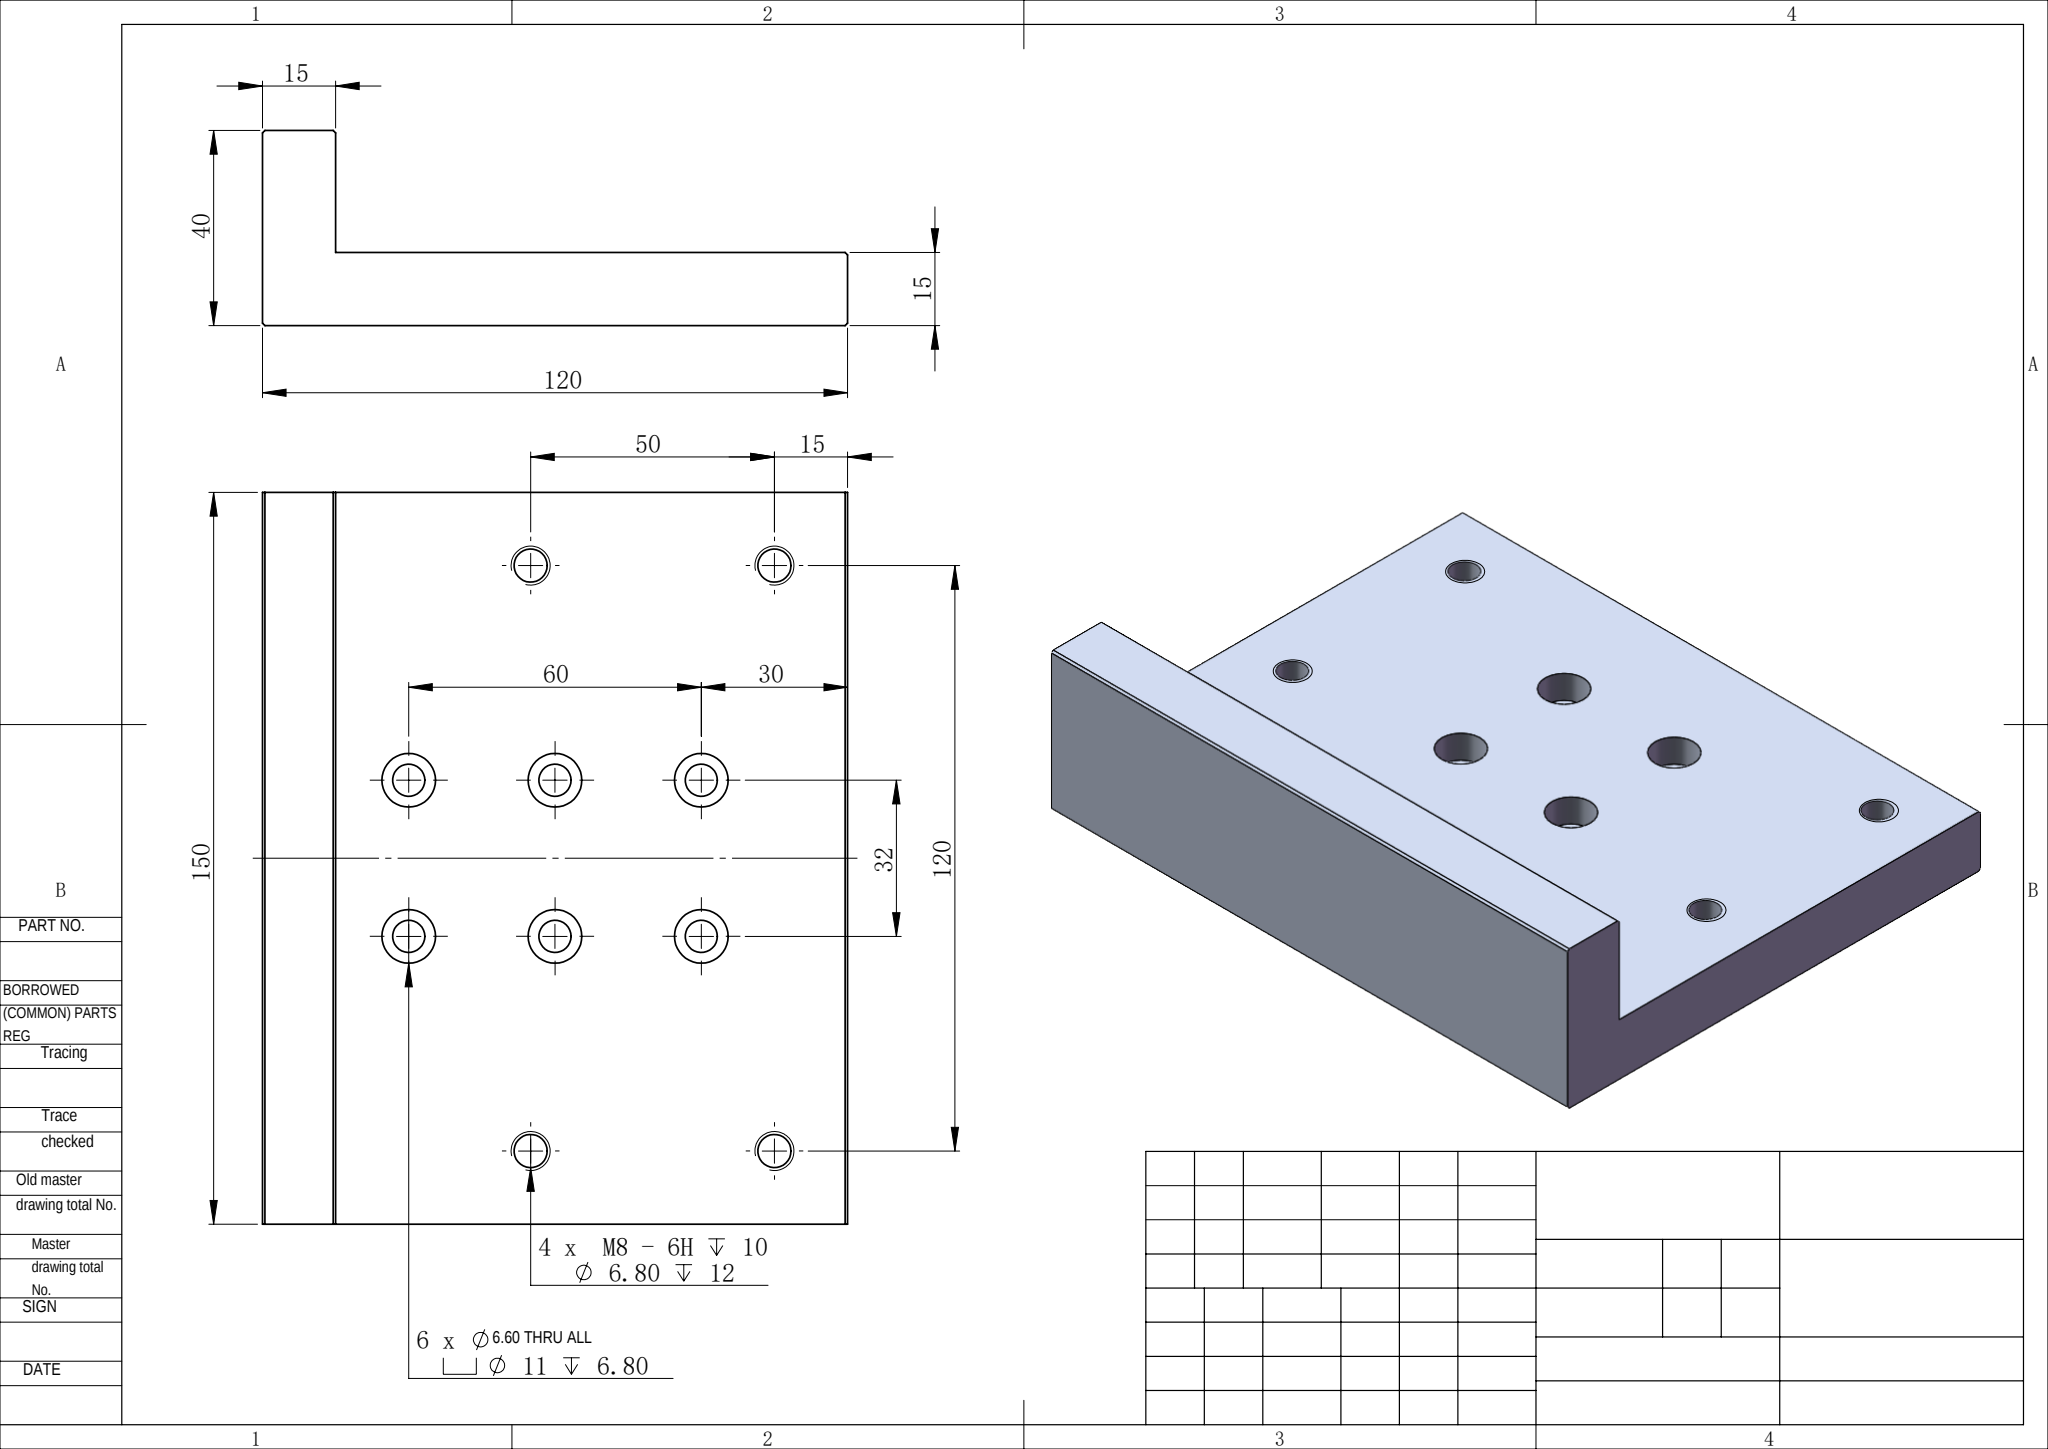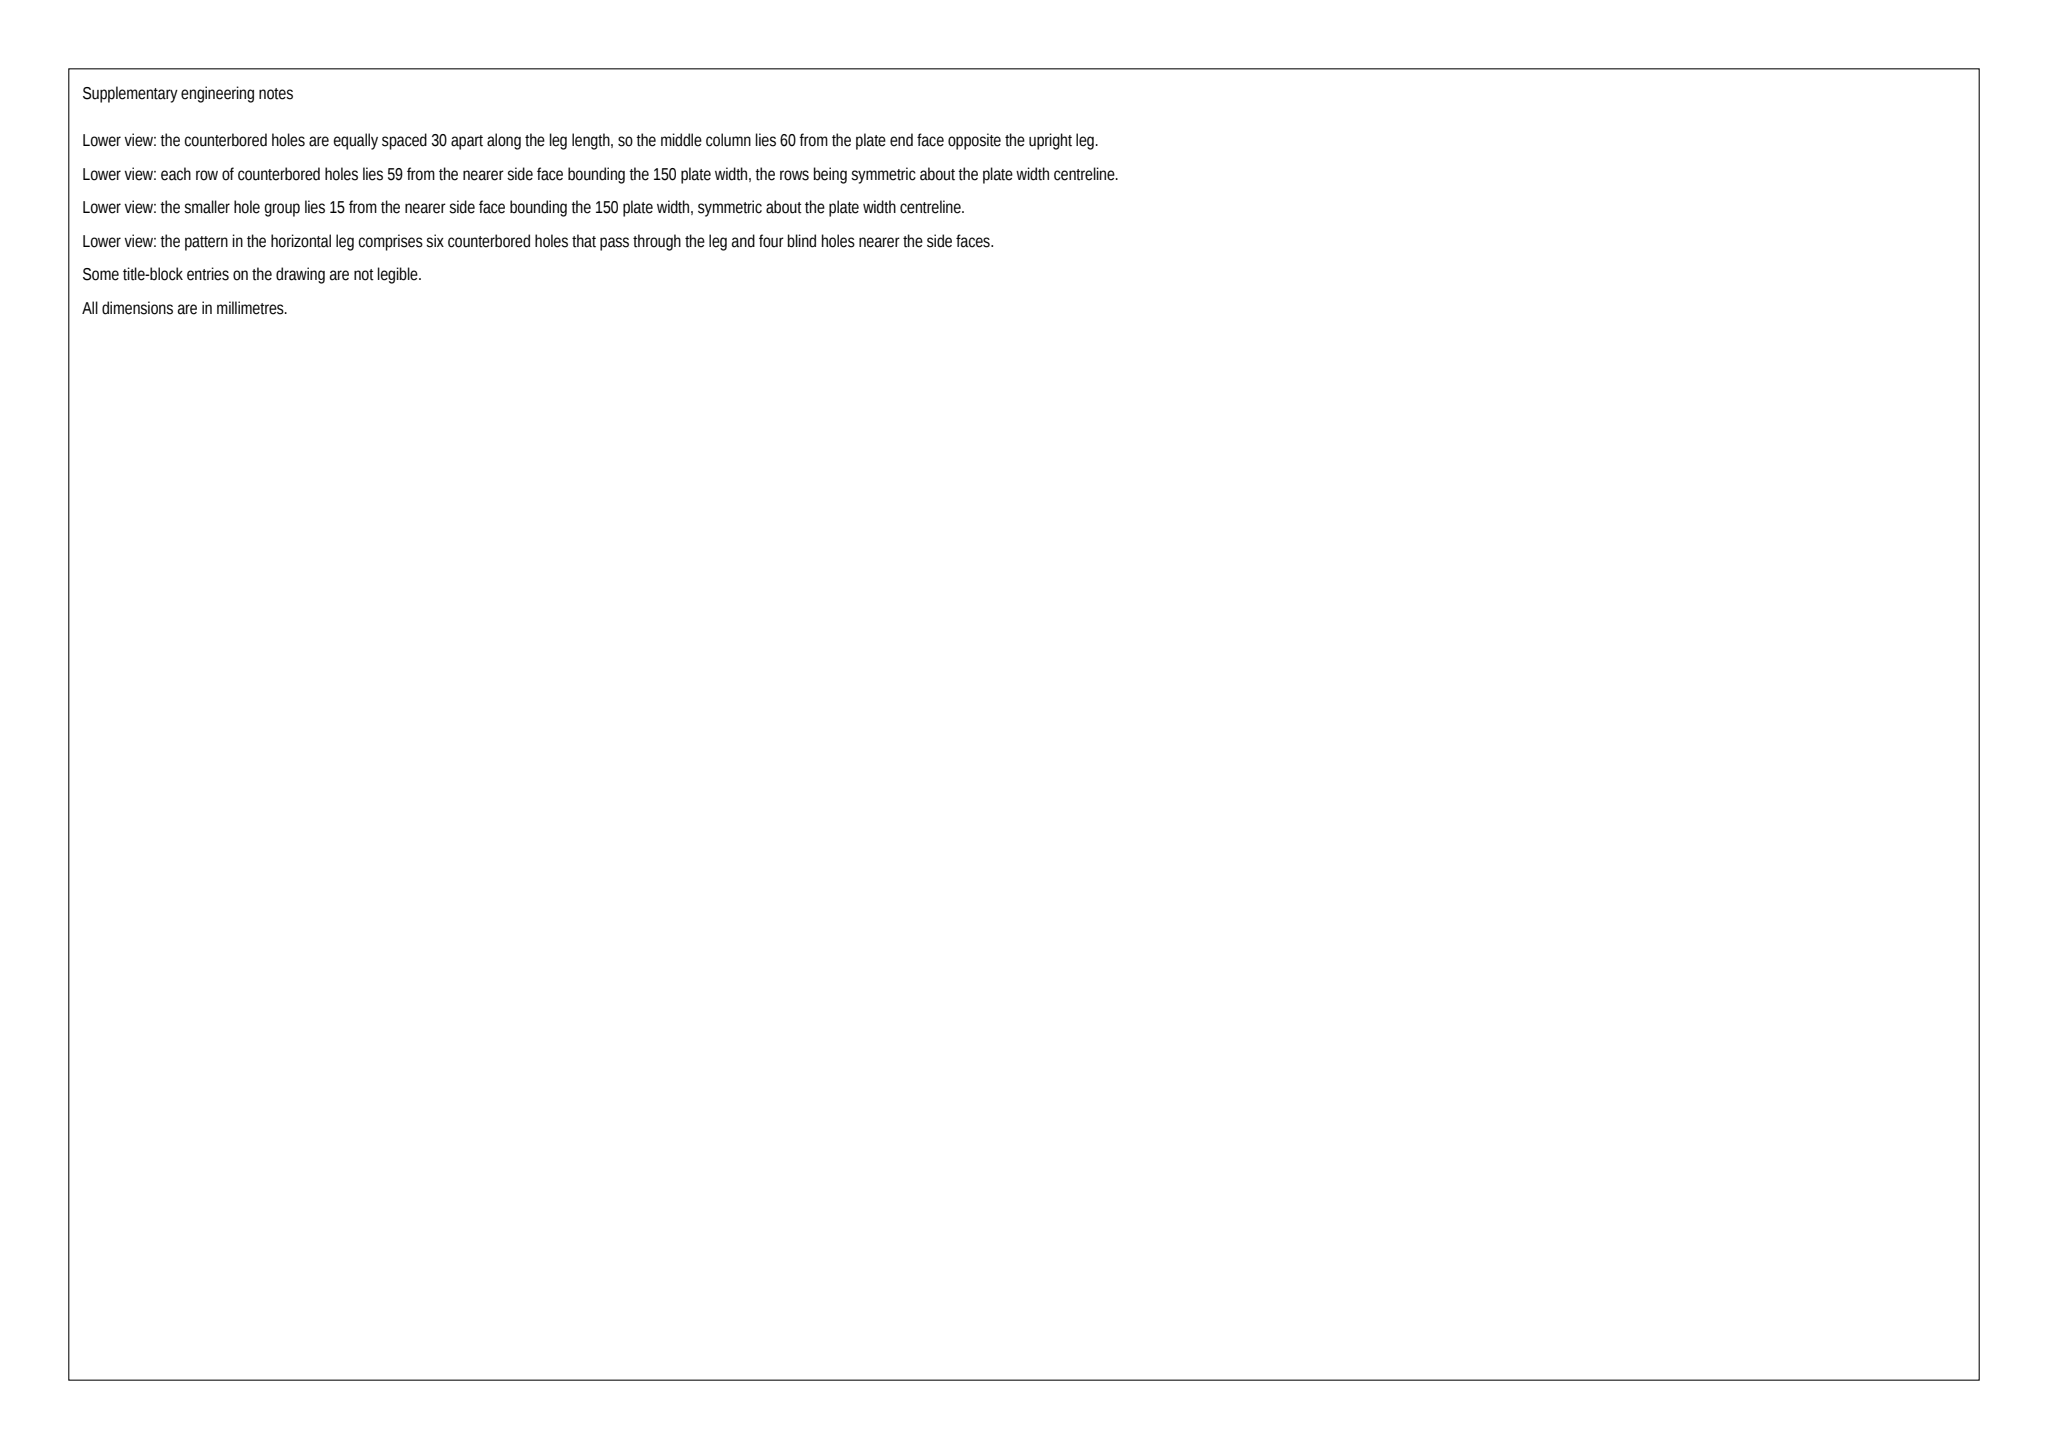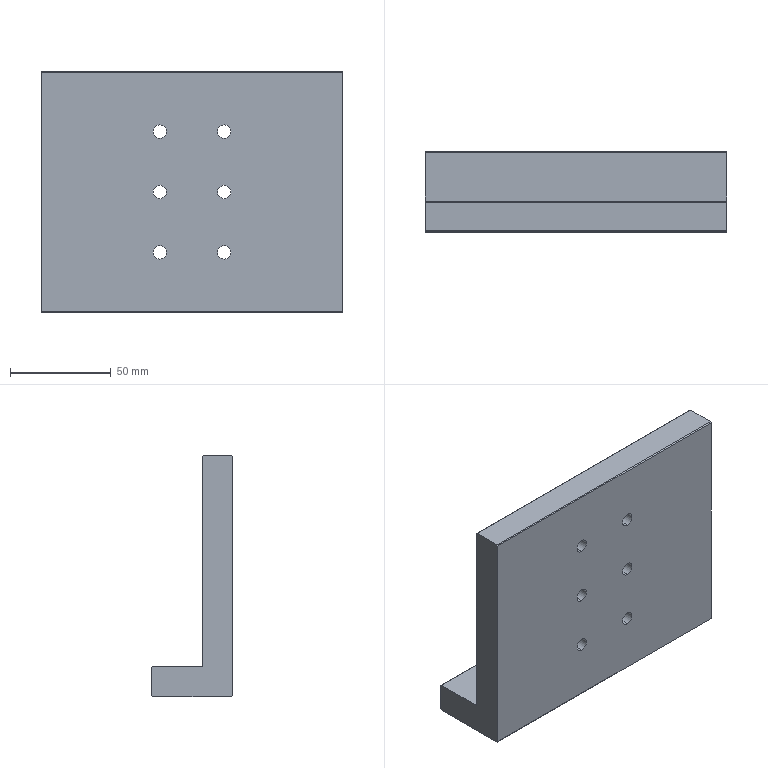Part | SolidWorks | mm | 1 solid | 59 faces | box 150 x 40 x 120 mm | volume 318754 mm3 | cylinder 32 | plane 19 | cone 8 | commonest cylinder face diameters 11 x12 6.6 x12 6.8 x8
Drawing notes:
4 x M8-6H: 15 FROM EA 150 EDGE, 120 APART | from the solid: Ø6.8 tapped-hole axes at x=15 and x=135 of 150 bbox; spacing 120
build123d program:
from build123d import *

# Parameters (mm, degrees)
BOSS_EXTRUDE1_DEPTH                               = 75
HOLE_SIZE_ACCORDING_TO_TYPE_1_OF_HEXA_D           = 6.6
HOLE_SIZE_ACCORDING_TO_TYPE_1_OF_HEXA_CBORE_D     = 11
HOLE_SIZE_ACCORDING_TO_TYPE_1_OF_HEXA_CBORE_DEPTH = 6.8
CHAMFER1_SIZE                                     = 0.5
M8_TAPPED_HOLE1_D                                 = 6.8
M8_TAPPED_HOLE1_DEPTH                             = 12
M8_TAPPED_HOLE1_TIP                               = 2.043


with BuildPart() as part:
    # Sketch1 → Boss-Extrude1 (new, symmetric)
    with BuildSketch(Plane(origin=(0, 0, 0), x_dir=(0, 0, -1), z_dir=(1, 0, 0))):
        Polygon((0, 0), (-120, 0), (-120, 15), (-15, 15), (-15, 40), (0, 40), align=None)
    extrude(amount=BOSS_EXTRUDE1_DEPTH, both=True)

    # Hole Size _ according to_ Type 1 of Hexa (through all)
    with Locations(Plane(origin=(0, 15, 0), x_dir=(1, 0, 0), z_dir=(0, 1, 0))):
        with Locations((-16, -30), (16, -90), (-16, -90), (16, -30), (-16, -60), (16, -60)):
            CounterBoreHole(HOLE_SIZE_ACCORDING_TO_TYPE_1_OF_HEXA_D / 2, HOLE_SIZE_ACCORDING_TO_TYPE_1_OF_HEXA_CBORE_D / 2, HOLE_SIZE_ACCORDING_TO_TYPE_1_OF_HEXA_CBORE_DEPTH)

    # Chamfer1
    chamfer1_edges = [part.edges().sort_by_distance(p)[0] for p in [
        (0, 0, 0),
        (0, 0, 120),
        (0, 15, 120),
        (0, 40, 15),
        (0, 40, 0),
    ]]
    chamfer(chamfer1_edges, length=CHAMFER1_SIZE)

    # M8 Tapped Hole1
    with Locations(Plane(origin=(0, 15, 0), x_dir=(1, 0, 0), z_dir=(0, 1, 0))):
        with Locations((-60, -55), (60, -105), (-60, -105), (60, -55)):
            Hole(M8_TAPPED_HOLE1_D / 2, depth=M8_TAPPED_HOLE1_DEPTH)
            with Locations((0, 0, -(M8_TAPPED_HOLE1_DEPTH + M8_TAPPED_HOLE1_TIP / 2))):  # 118° drill point
                Cone(0, M8_TAPPED_HOLE1_D / 2, M8_TAPPED_HOLE1_TIP, mode=Mode.SUBTRACT)


solid = part.part